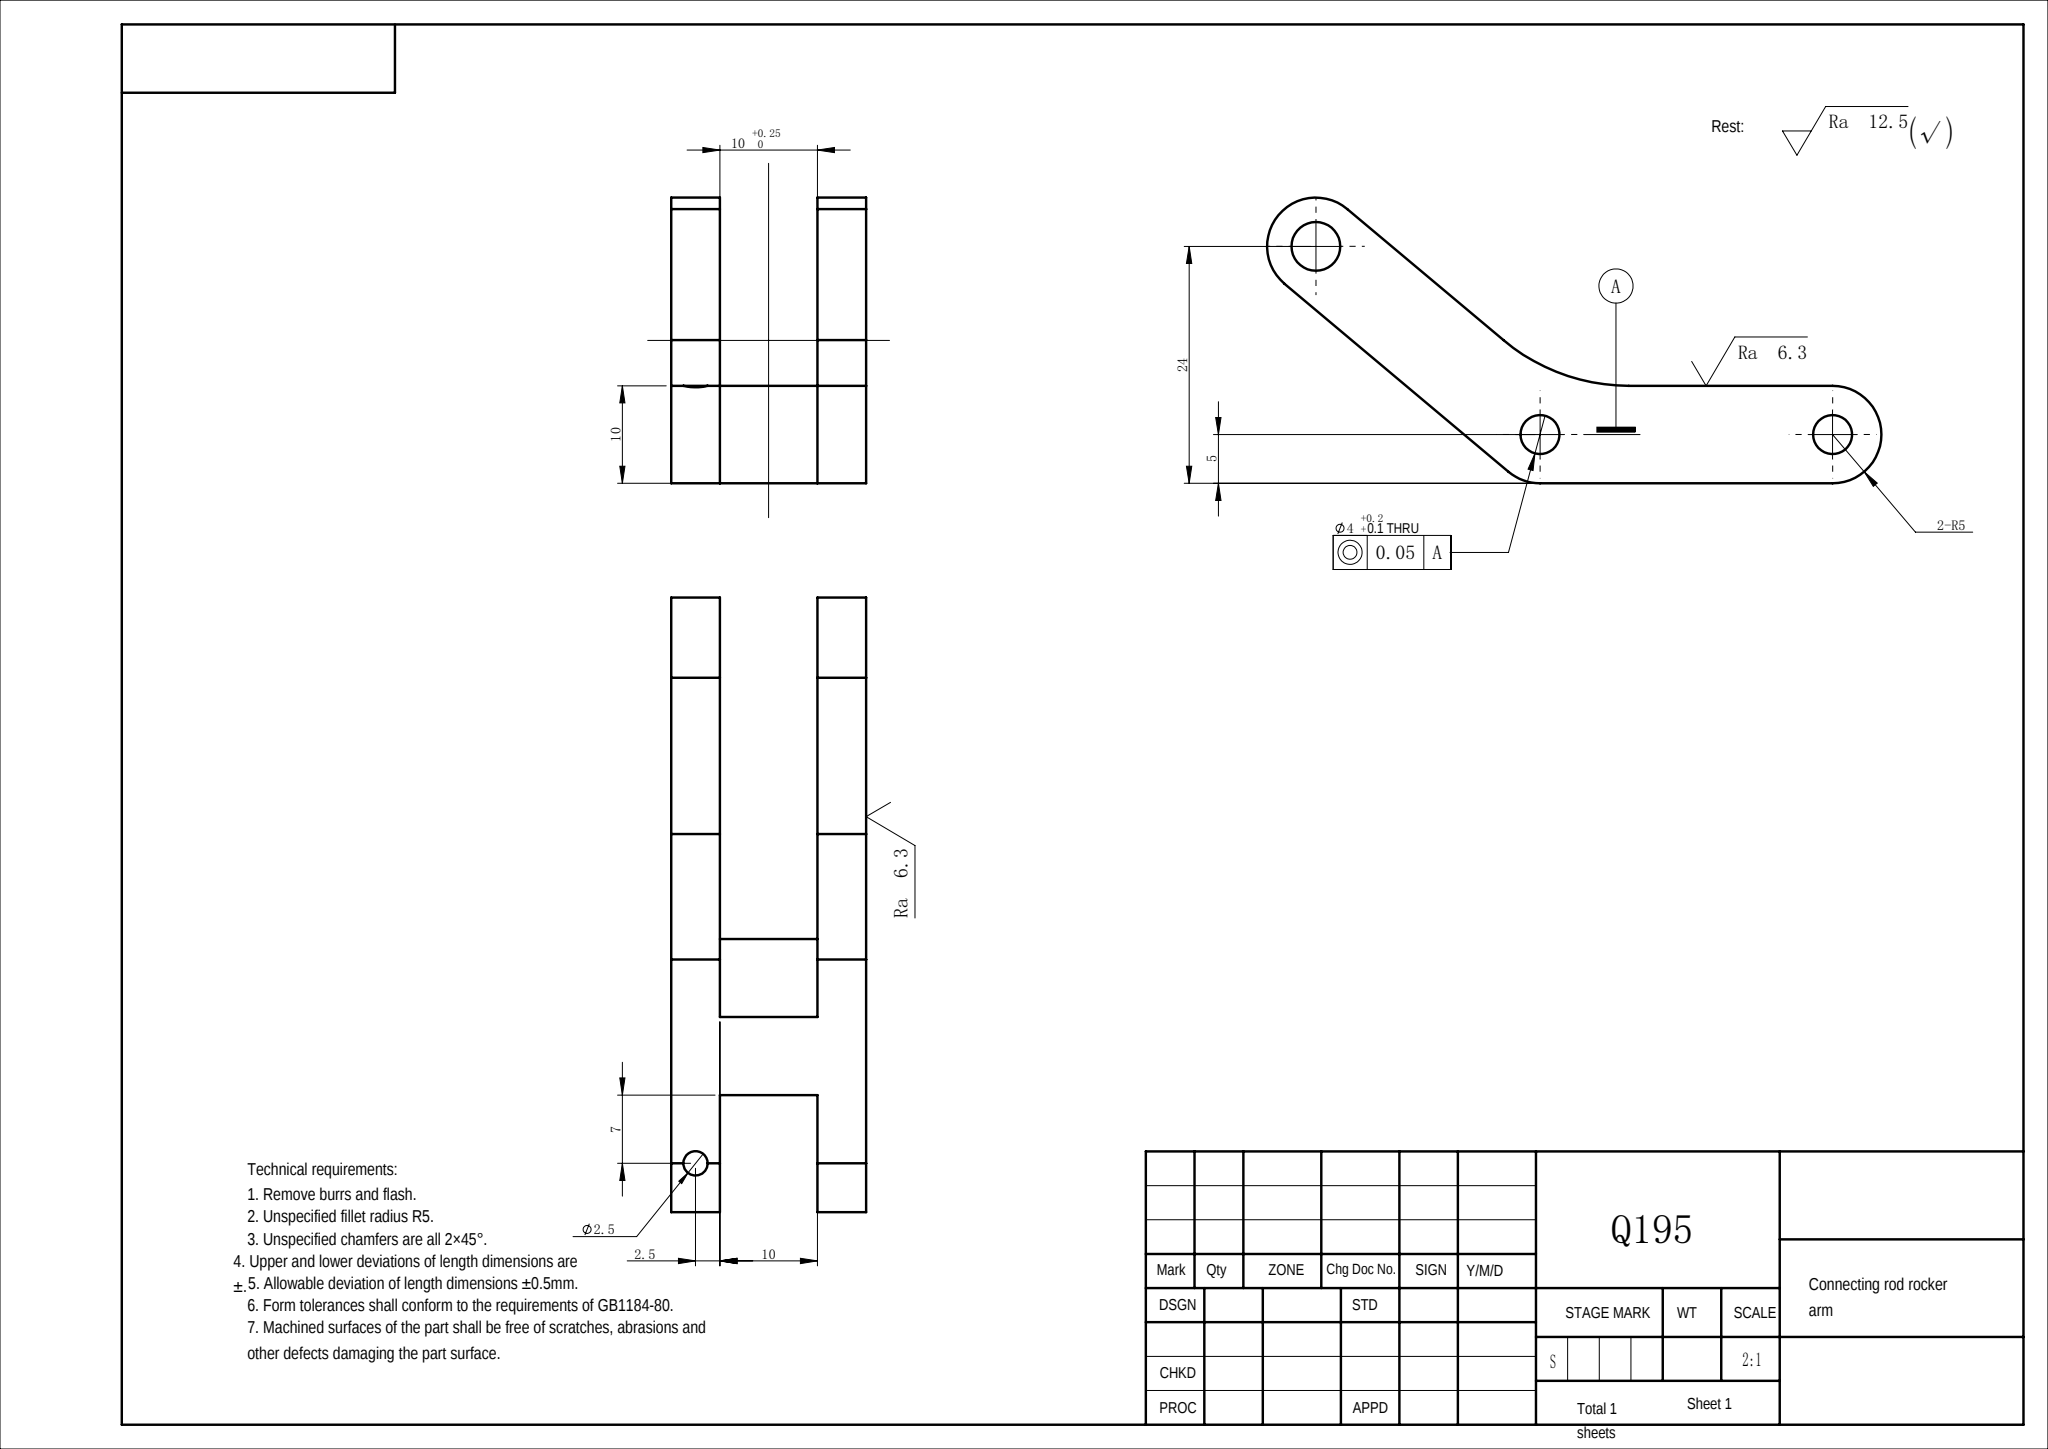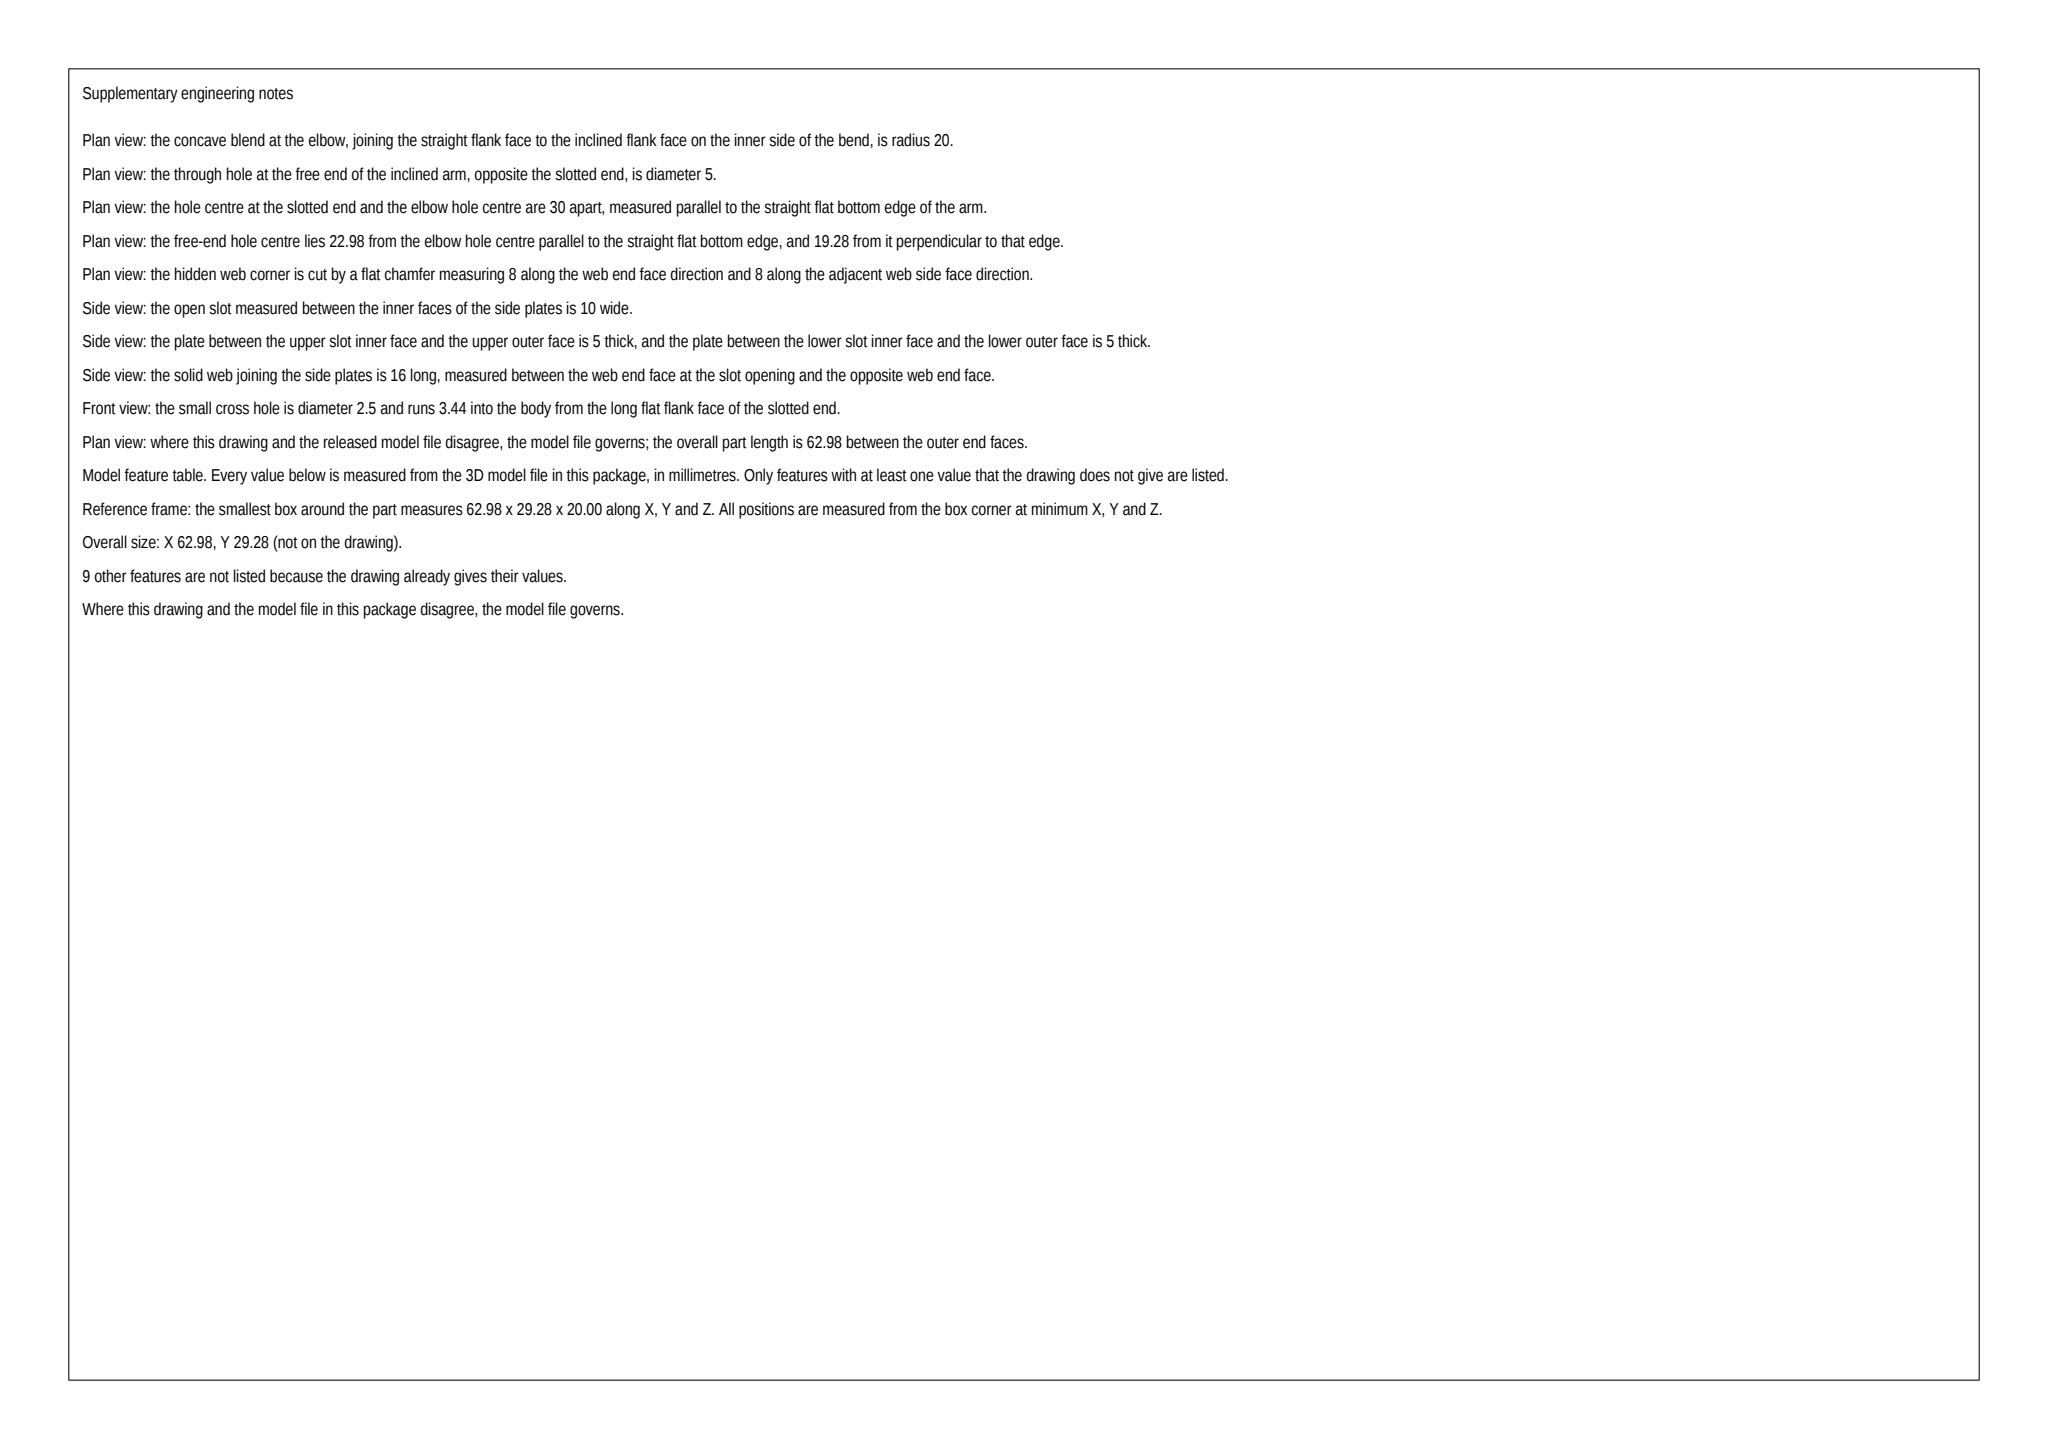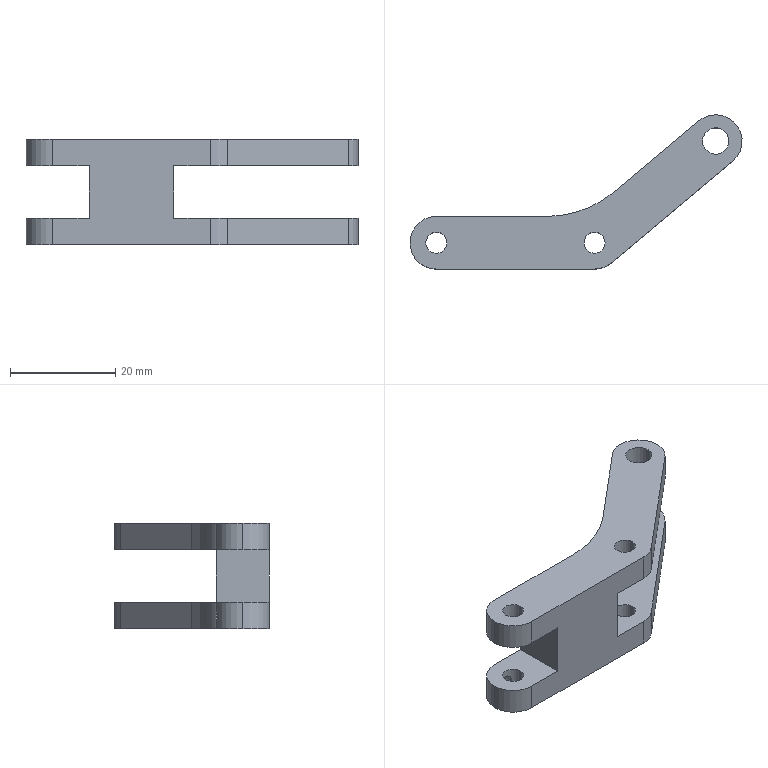Part | SolidWorks | drawing in inches | material Q195 | 1 solid | 39 faces | box 62.98 x 29.28 x 20 mm | volume 7658 mm3 | cylinder 24 | plane 15 | commonest cylinder face diameters 10 x8 4 x8 5 x4 2.5 x2 40 x2